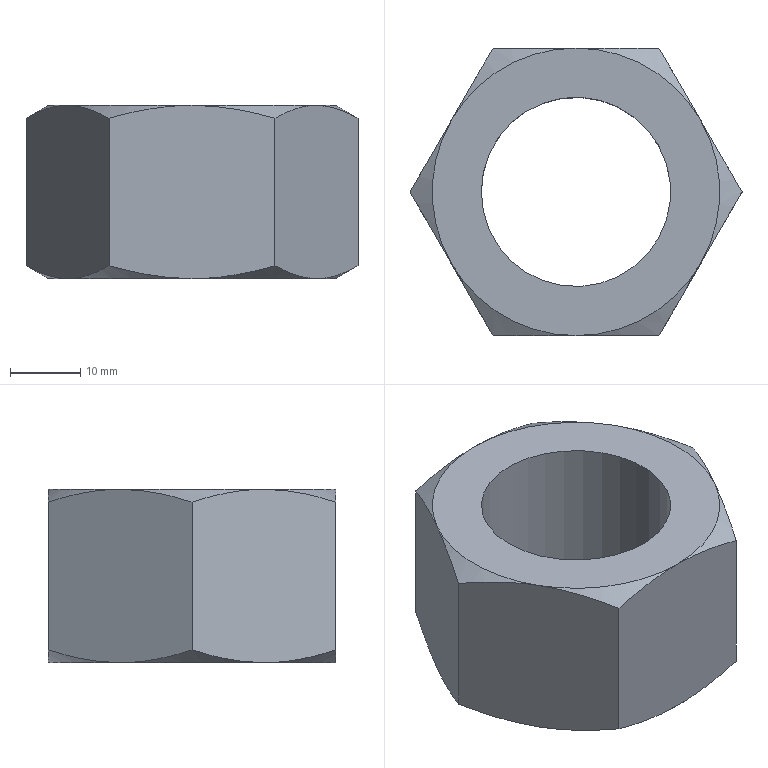Component | NX | NUT_M27 | 1 solid | 21 faces | volume 21664 mm3 | cone 12 | plane 8 | cylinder 1 | commonest cylinder face diameters 27 x1